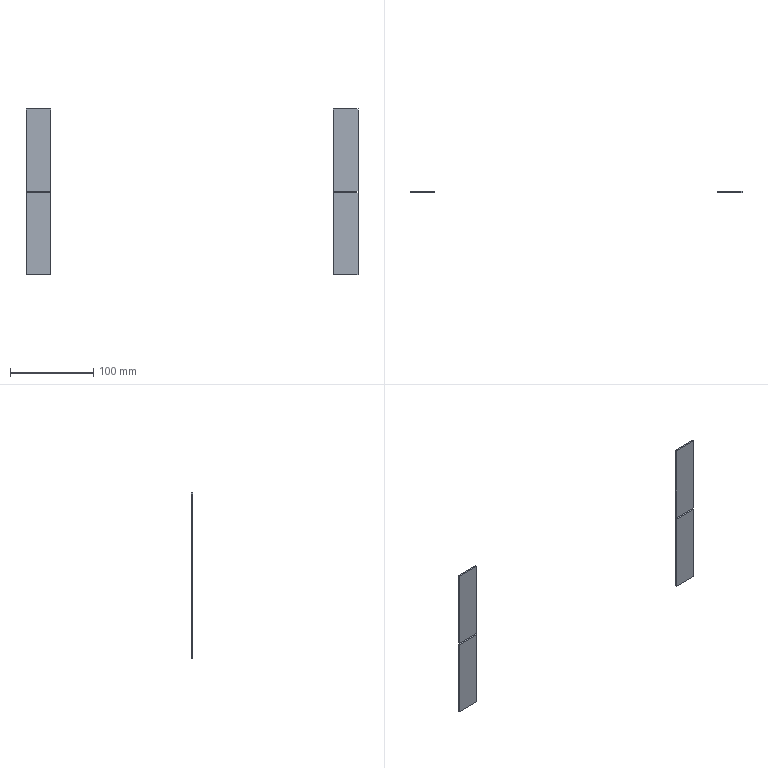Component | NX | DATUM | 4 solids | 24 faces | volume 23748 mm3 | plane 24